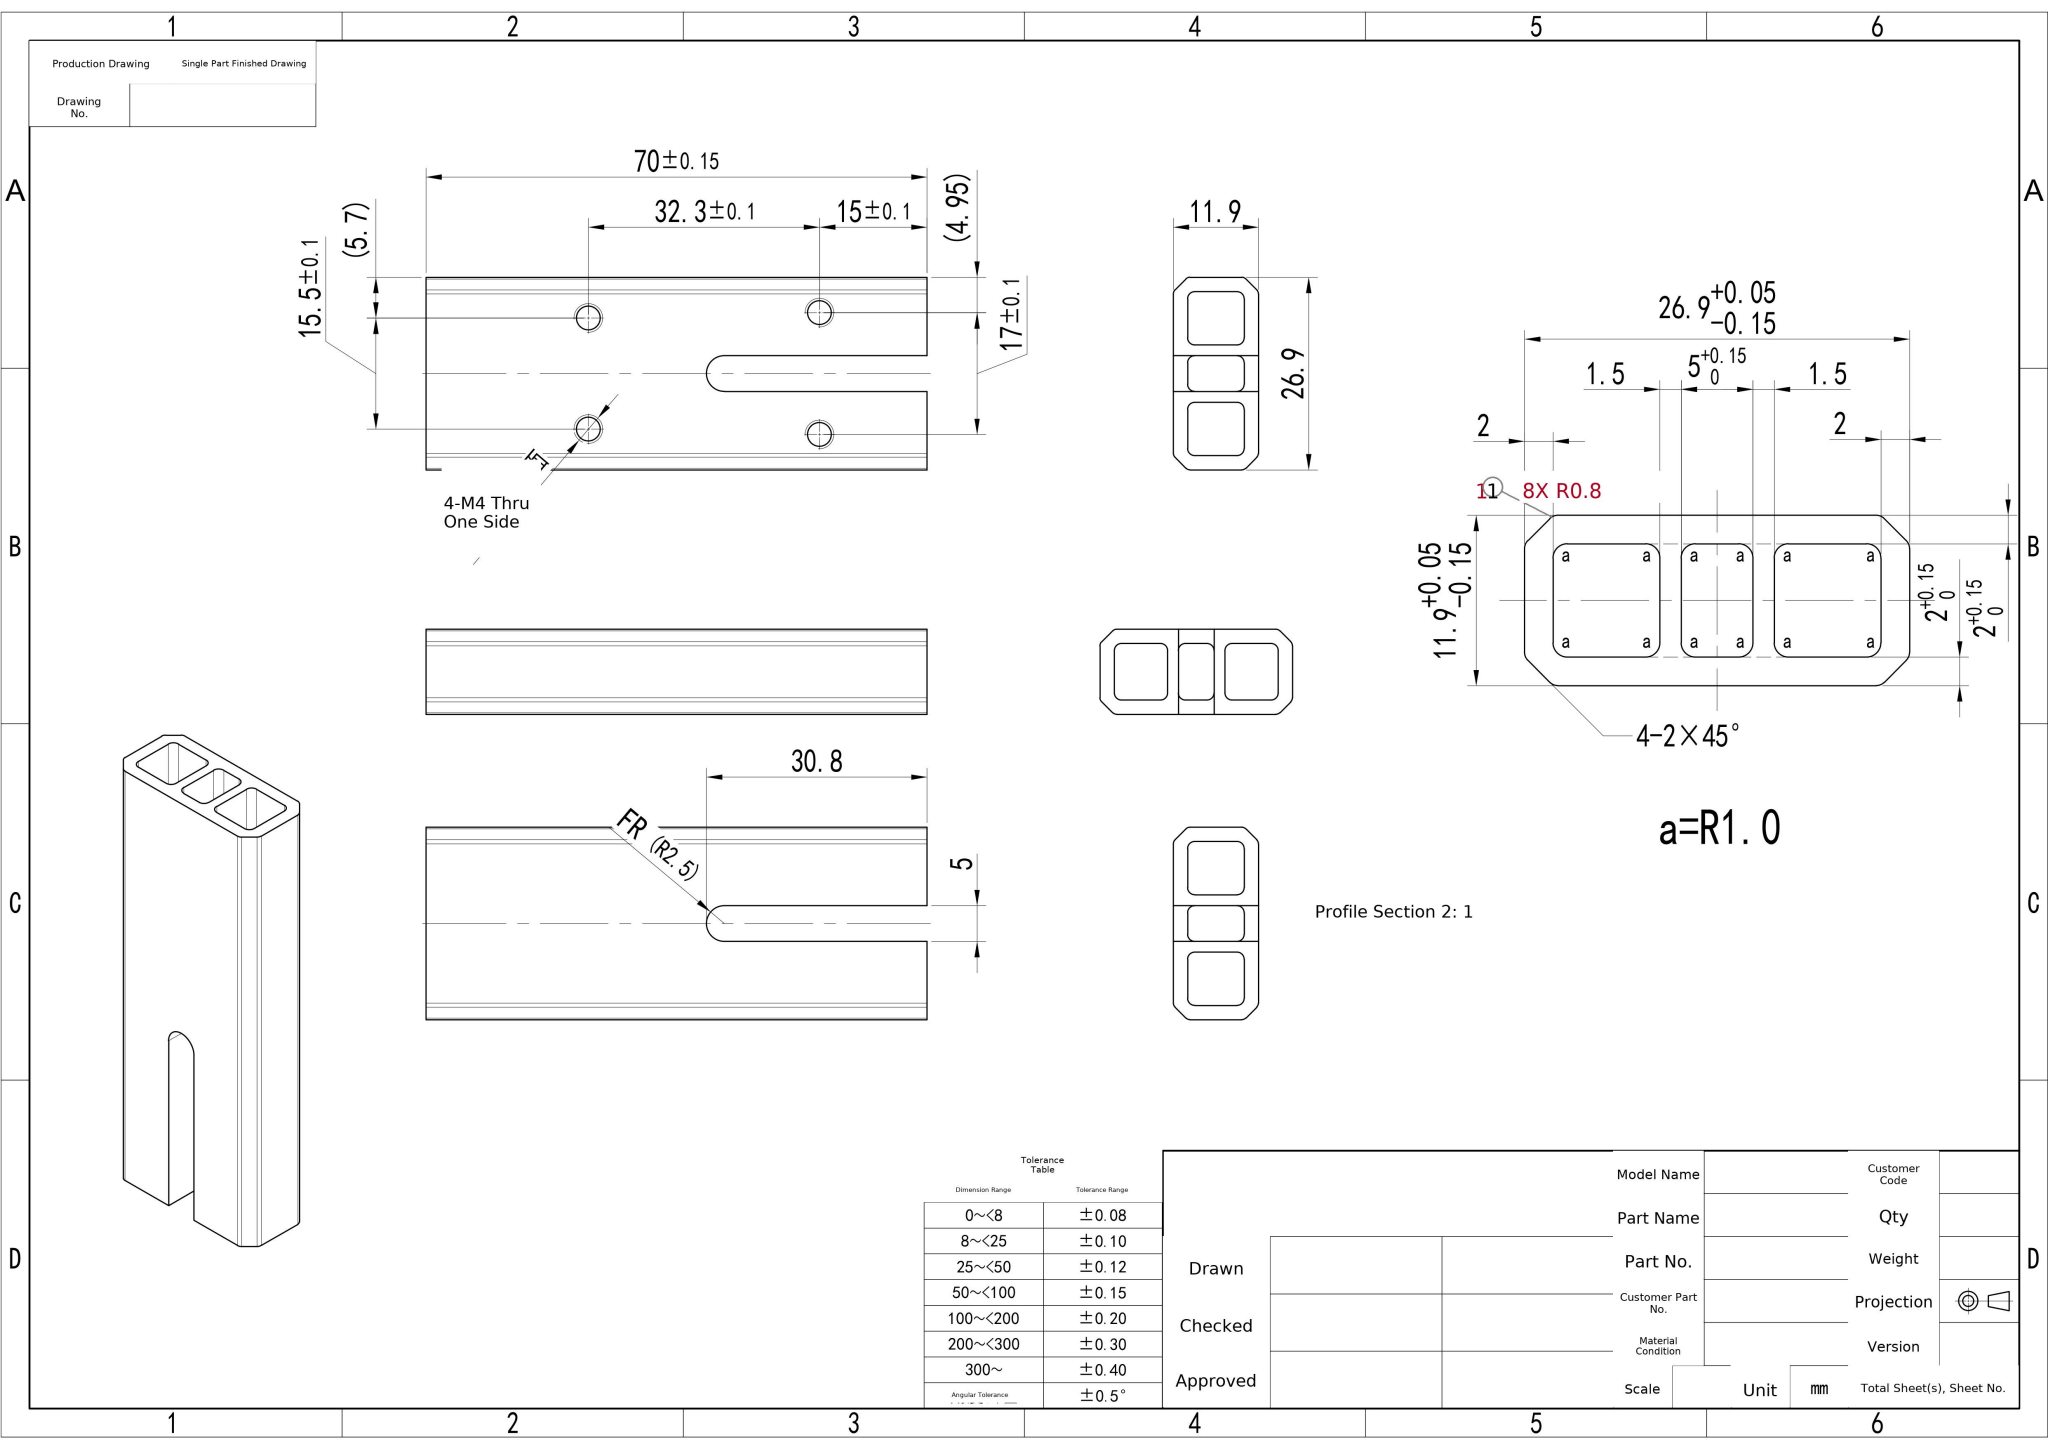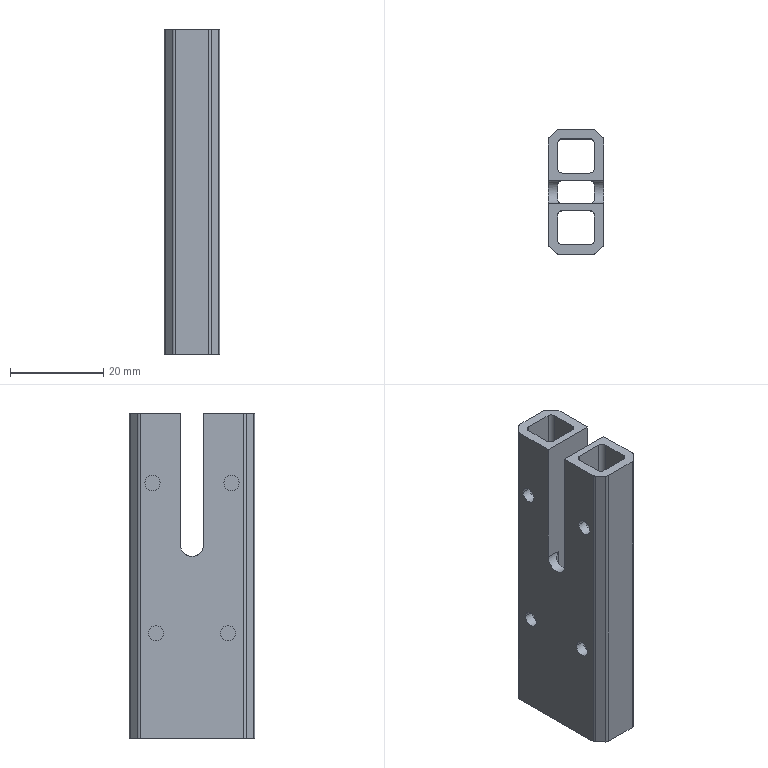Part | SolidWorks | mm | 1 solid | 53 faces | box 11.9 x 26.9 x 70 mm | volume 10317 mm3 | cylinder 30 | plane 23 | commonest cylinder face diameters 2 x12 3.3 x8 1.6 x8 5 x2